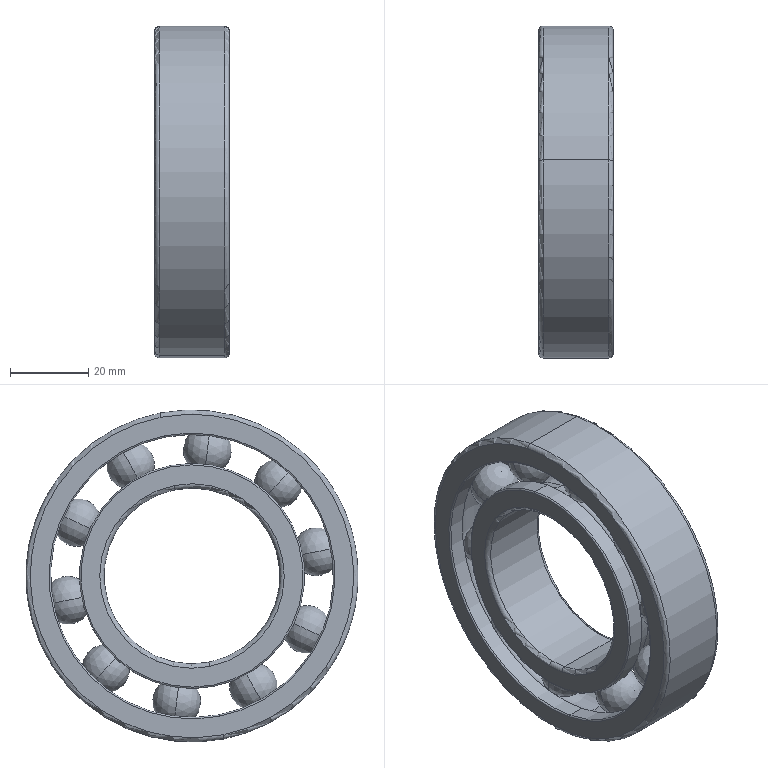Component | SolidWorks | bearing dan rumahan assembly-2_SKF_6209-3 | 12 solids | 58 faces | volume 51525 mm3 | torus 22 | sphere 20 | cylinder 12 | plane 4 | commonest cylinder face diameters 57.6 x4 72.4 x4 45 x2 85 x2